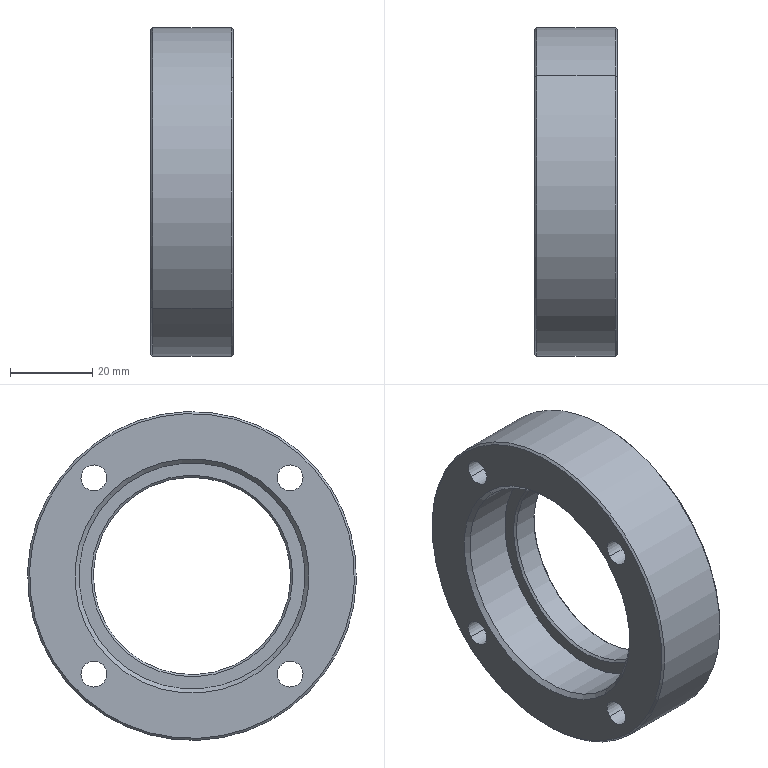Component | SolidWorks | LowerSideBeltXG-XG1-1_GB6006BearingHousingXG-XG1-1 | 1 solid | 39 faces | box 20 x 80 x 80 mm | volume 52764 mm3 | cylinder 22 | cone 10 | plane 7 | commonest cylinder face diameters 11 x8 6.3 x8 80 x2 55 x2 48 x2
STEP:
#1=COLOUR_RGB('',0.7922,0.8196,0.9333);
#2=FILL_AREA_STYLE_COLOUR('',#1);
#3=FILL_AREA_STYLE('',(#2));
#4=SURFACE_STYLE_FILL_AREA(#3);
#5=SURFACE_SIDE_STYLE('',(#4));
#6=SURFACE_STYLE_USAGE(.BOTH.,#5);
#7=PRESENTATION_STYLE_ASSIGNMENT((#6));
#8=CARTESIAN_POINT('',(-12.41,25.372,5.254));
#9=VERTEX_POINT('',#8);
#10=CARTESIAN_POINT('',(-12.41,23.841,3.723));
#11=VERTEX_POINT('',#10);
#12=CARTESIAN_POINT('',(-12.41,24.606,4.488));
#13=DIRECTION('',(-1.,-0.,-0.));
#14=DIRECTION('',(0.,-0.7071,-0.7071));
#15=AXIS2_PLACEMENT_3D('',#12,#13,#14);
#16=CIRCLE('',#15,1.083);
#17=EDGE_CURVE('',#9,#11,#16,.T.);
#18=ORIENTED_EDGE('',*,*,#17,.F.);
#19=CARTESIAN_POINT('',(-12.45,25.4,5.282));
#20=VERTEX_POINT('',#19);
#21=CARTESIAN_POINT('',(-12.45,25.4,5.282));
#22=DIRECTION('',(-0.7071,0.5,0.5));
#23=VECTOR('',#22,39.37);
#24=LINE('',#21,#23);
#25=EDGE_CURVE('',#9,#20,#24,.T.);
#26=ORIENTED_EDGE('',*,*,#25,.T.);
#27=CARTESIAN_POINT('',(-12.45,23.813,3.695));
#28=VERTEX_POINT('',#27);
#29=CARTESIAN_POINT('',(-12.45,24.606,4.488));
#30=DIRECTION('',(1.,0.,0.));
#31=DIRECTION('',(0.,-0.7071,-0.7071));
#32=AXIS2_PLACEMENT_3D('',#29,#30,#31);
#33=CIRCLE('',#32,1.122);
#34=EDGE_CURVE('',#28,#20,#33,.T.);
#35=ORIENTED_EDGE('',*,*,#34,.F.);
#36=CARTESIAN_POINT('',(-12.45,23.813,3.695));
#37=DIRECTION('',(-0.7071,-0.5,-0.5));
#38=VECTOR('',#37,39.37);
#39=LINE('',#36,#38);
#40=EDGE_CURVE('',#11,#28,#39,.T.);
#41=ORIENTED_EDGE('',*,*,#40,.F.);
#42=EDGE_LOOP('',(#18,#26,#35,#41));
#43=FACE_OUTER_BOUND('',#42,.T.);
#44=CARTESIAN_POINT('',(-12.45,24.606,4.488));
#45=DIRECTION('',(-1.,-0.,-0.));
#46=DIRECTION('',(0.,-0.7071,-0.7071));
#47=AXIS2_PLACEMENT_3D('',#44,#45,#46);
#48=CONICAL_SURFACE('',#47,1.122,0.7854);
#49=ADVANCED_FACE('',(#43),#48,.F.);
#50=CARTESIAN_POINT('',(-11.918,25.274,5.156));
#51=VERTEX_POINT('',#50);
#52=CARTESIAN_POINT('',(-11.918,23.938,3.82));
#53=VERTEX_POINT('',#52);
#54=CARTESIAN_POINT('',(-11.918,24.606,4.488));
#55=DIRECTION('',(-1.,-0.,-0.));
#56=DIRECTION('',(0.,-0.7071,-0.7071));
#57=AXIS2_PLACEMENT_3D('',#54,#55,#56);
#58=CIRCLE('',#57,0.9449);
#59=EDGE_CURVE('',#51,#53,#58,.T.);
#60=ORIENTED_EDGE('',*,*,#59,.F.);
#61=CARTESIAN_POINT('',(-11.938,25.288,5.17));
#62=VERTEX_POINT('',#61);
#63=CARTESIAN_POINT('',(-11.938,25.288,5.17));
#64=DIRECTION('',(-0.7071,0.5,0.5));
#65=VECTOR('',#64,39.37);
#66=LINE('',#63,#65);
#67=EDGE_CURVE('',#51,#62,#66,.T.);
#68=ORIENTED_EDGE('',*,*,#67,.T.);
#69=CARTESIAN_POINT('',(-11.938,23.924,3.806));
#70=VERTEX_POINT('',#69);
#71=CARTESIAN_POINT('',(-11.938,24.606,4.488));
#72=DIRECTION('',(1.,0.,0.));
#73=DIRECTION('',(0.,-0.7071,-0.7071));
#74=AXIS2_PLACEMENT_3D('',#71,#72,#73);
#75=CIRCLE('',#74,0.9646);
#76=EDGE_CURVE('',#70,#62,#75,.T.);
#77=ORIENTED_EDGE('',*,*,#76,.F.);
#78=CARTESIAN_POINT('',(-11.938,23.924,3.806));
#79=DIRECTION('',(-0.7071,-0.5,-0.5));
#80=VECTOR('',#79,39.37);
#81=LINE('',#78,#80);
#82=EDGE_CURVE('',#53,#70,#81,.T.);
#83=ORIENTED_EDGE('',*,*,#82,.F.);
#84=EDGE_LOOP('',(#60,#68,#77,#83));
#85=FACE_OUTER_BOUND('',#84,.T.);
#86=CARTESIAN_POINT('',(-11.938,24.606,4.488));
#87=DIRECTION('',(-1.,-0.,-0.));
#88=DIRECTION('',(0.,-0.7071,-0.7071));
#89=AXIS2_PLACEMENT_3D('',#86,#87,#88);
#90=CONICAL_SURFACE('',#89,0.9646,0.7854);
#91=ADVANCED_FACE('',(#85),#90,.F.);
#92=CARTESIAN_POINT('',(-11.682,23.938,3.82));
#93=VERTEX_POINT('',#92);
#94=CARTESIAN_POINT('',(-11.682,25.274,5.156));
#95=VERTEX_POINT('',#94);
#96=CARTESIAN_POINT('',(-11.682,24.606,4.488));
#97=DIRECTION('',(1.,0.,0.));
#98=DIRECTION('',(-0.,0.7071,0.7071));
#99=AXIS2_PLACEMENT_3D('',#96,#97,#98);
#100=CIRCLE('',#99,0.9449);
#101=EDGE_CURVE('',#93,#95,#100,.T.);
#102=ORIENTED_EDGE('',*,*,#101,.F.);
#103=CARTESIAN_POINT('',(-11.662,23.924,3.806));
#104=VERTEX_POINT('',#103);
#105=CARTESIAN_POINT('',(-11.682,23.938,3.82));
#106=DIRECTION('',(0.7071,-0.5,-0.5));
#107=VECTOR('',#106,39.37);
#108=LINE('',#105,#107);
#109=EDGE_CURVE('',#93,#104,#108,.T.);
#110=ORIENTED_EDGE('',*,*,#109,.T.);
#111=CARTESIAN_POINT('',(-11.662,25.288,5.17));
#112=VERTEX_POINT('',#111);
#113=CARTESIAN_POINT('',(-11.662,24.606,4.488));
#114=DIRECTION('',(-1.,-0.,-0.));
#115=DIRECTION('',(-0.,0.7071,0.7071));
#116=AXIS2_PLACEMENT_3D('',#113,#114,#115);
#117=CIRCLE('',#116,0.9646);
#118=EDGE_CURVE('',#112,#104,#117,.T.);
#119=ORIENTED_EDGE('',*,*,#118,.F.);
#120=CARTESIAN_POINT('',(-11.682,25.274,5.156));
#121=DIRECTION('',(0.7071,0.5,0.5));
#122=VECTOR('',#121,39.37);
#123=LINE('',#120,#122);
#124=EDGE_CURVE('',#95,#112,#123,.T.);
#125=ORIENTED_EDGE('',*,*,#124,.F.);
#126=EDGE_LOOP('',(#102,#110,#119,#125));
#127=FACE_OUTER_BOUND('',#126,.T.);
#128=CARTESIAN_POINT('',(-11.682,24.606,4.488));
#129=DIRECTION('',(1.,0.,0.));
#130=DIRECTION('',(-0.,0.7071,0.7071));
#131=AXIS2_PLACEMENT_3D('',#128,#129,#130);
#132=CONICAL_SURFACE('',#131,0.9449,0.7854);
#133=ADVANCED_FACE('',(#127),#132,.F.);
#134=CARTESIAN_POINT('',(-11.662,25.706,5.588));
#135=VERTEX_POINT('',#134);
#136=CARTESIAN_POINT('',(-11.662,23.507,3.389));
#137=VERTEX_POINT('',#136);
#138=CARTESIAN_POINT('',(-11.662,24.606,4.488));
#139=DIRECTION('',(1.,0.,0.));
#140=DIRECTION('',(-0.,0.7071,0.7071));
#141=AXIS2_PLACEMENT_3D('',#138,#139,#140);
#142=CIRCLE('',#141,1.555);
#143=EDGE_CURVE('',#135,#137,#142,.T.);
#144=ORIENTED_EDGE('',*,*,#143,.F.);
#145=CARTESIAN_POINT('',(-11.682,25.72,5.602));
#146=VERTEX_POINT('',#145);
#147=CARTESIAN_POINT('',(-11.662,25.706,5.588));
#148=DIRECTION('',(-0.7071,0.5,0.5));
#149=VECTOR('',#148,39.37);
#150=LINE('',#147,#149);
#151=EDGE_CURVE('',#135,#146,#150,.T.);
#152=ORIENTED_EDGE('',*,*,#151,.T.);
#153=CARTESIAN_POINT('',(-11.682,23.493,3.375));
#154=VERTEX_POINT('',#153);
#155=CARTESIAN_POINT('',(-11.682,24.606,4.488));
#156=DIRECTION('',(-1.,-0.,-0.));
#157=DIRECTION('',(-0.,0.7071,0.7071));
#158=AXIS2_PLACEMENT_3D('',#155,#156,#157);
#159=CIRCLE('',#158,1.575);
#160=EDGE_CURVE('',#154,#146,#159,.T.);
#161=ORIENTED_EDGE('',*,*,#160,.F.);
#162=CARTESIAN_POINT('',(-11.662,23.507,3.389));
#163=DIRECTION('',(-0.7071,-0.5,-0.5));
#164=VECTOR('',#163,39.37);
#165=LINE('',#162,#164);
#166=EDGE_CURVE('',#137,#154,#165,.T.);
#167=ORIENTED_EDGE('',*,*,#166,.F.);
#168=EDGE_LOOP('',(#144,#152,#161,#167));
#169=FACE_OUTER_BOUND('',#168,.T.);
#170=CARTESIAN_POINT('',(-11.662,24.606,4.488));
#171=DIRECTION('',(-1.,-0.,-0.));
#172=DIRECTION('',(0.,-0.7071,-0.7071));
#173=AXIS2_PLACEMENT_3D('',#170,#171,#172);
#174=CONICAL_SURFACE('',#173,1.555,0.7854);
#175=ADVANCED_FACE('',(#169),#174,.T.);
#176=CARTESIAN_POINT('',(-12.45,23.507,3.389));
#177=VERTEX_POINT('',#176);
#178=CARTESIAN_POINT('',(-12.45,25.706,5.588));
#179=VERTEX_POINT('',#178);
#180=CARTESIAN_POINT('',(-12.45,24.606,4.488));
#181=DIRECTION('',(-1.,-0.,-0.));
#182=DIRECTION('',(0.,-0.7071,-0.7071));
#183=AXIS2_PLACEMENT_3D('',#180,#181,#182);
#184=CIRCLE('',#183,1.555);
#185=EDGE_CURVE('',#177,#179,#184,.T.);
#186=ORIENTED_EDGE('',*,*,#185,.F.);
#187=CARTESIAN_POINT('',(-12.43,23.493,3.375));
#188=VERTEX_POINT('',#187);
#189=CARTESIAN_POINT('',(-12.43,23.493,3.375));
#190=DIRECTION('',(0.7071,-0.5,-0.5));
#191=VECTOR('',#190,39.37);
#192=LINE('',#189,#191);
#193=EDGE_CURVE('',#177,#188,#192,.T.);
#194=ORIENTED_EDGE('',*,*,#193,.T.);
#195=CARTESIAN_POINT('',(-12.43,25.72,5.602));
#196=VERTEX_POINT('',#195);
#197=CARTESIAN_POINT('',(-12.43,24.606,4.488));
#198=DIRECTION('',(1.,0.,0.));
#199=DIRECTION('',(0.,-0.7071,-0.7071));
#200=AXIS2_PLACEMENT_3D('',#197,#198,#199);
#201=CIRCLE('',#200,1.575);
#202=EDGE_CURVE('',#196,#188,#201,.T.);
#203=ORIENTED_EDGE('',*,*,#202,.F.);
#204=CARTESIAN_POINT('',(-12.43,25.72,5.602));
#205=DIRECTION('',(0.7071,0.5,0.5));
#206=VECTOR('',#205,39.37);
#207=LINE('',#204,#206);
#208=EDGE_CURVE('',#179,#196,#207,.T.);
#209=ORIENTED_EDGE('',*,*,#208,.F.);
#210=EDGE_LOOP('',(#186,#194,#203,#209));
#211=FACE_OUTER_BOUND('',#210,.T.);
#212=CARTESIAN_POINT('',(-12.43,24.606,4.488));
#213=DIRECTION('',(1.,0.,0.));
#214=DIRECTION('',(-0.,0.7071,0.7071));
#215=AXIS2_PLACEMENT_3D('',#212,#213,#214);
#216=CONICAL_SURFACE('',#215,1.575,0.7854);
#217=ADVANCED_FACE('',(#211),#216,.T.);
#218=CARTESIAN_POINT('',(-11.898,25.393,3.702));
#219=VERTEX_POINT('',#218);
#220=CARTESIAN_POINT('',(-11.898,25.699,3.396));
#221=VERTEX_POINT('',#220);
#222=CARTESIAN_POINT('',(-11.898,25.546,3.549));
#223=DIRECTION('',(1.,0.,-0.));
#224=DIRECTION('',(0.,0.7071,-0.7071));
#225=AXIS2_PLACEMENT_3D('',#222,#223,#224);
#226=CIRCLE('',#225,0.2165);
#227=EDGE_CURVE('',#219,#221,#226,.T.);
#228=ORIENTED_EDGE('',*,*,#227,.F.);
#229=CARTESIAN_POINT('',(-11.662,25.393,3.702));
#230=VERTEX_POINT('',#229);
#231=CARTESIAN_POINT('',(-11.662,25.393,3.702));
#232=DIRECTION('',(1.,0.,-0.));
#233=VECTOR('',#232,39.37);
#234=LINE('',#231,#233);
#235=EDGE_CURVE('',#219,#230,#234,.T.);
#236=ORIENTED_EDGE('',*,*,#235,.T.);
#237=CARTESIAN_POINT('',(-11.662,25.699,3.396));
#238=VERTEX_POINT('',#237);
#239=CARTESIAN_POINT('',(-11.662,25.546,3.549));
#240=DIRECTION('',(1.,0.,-0.));
#241=DIRECTION('',(0.,0.7071,-0.7071));
#242=AXIS2_PLACEMENT_3D('',#239,#240,#241);
#243=CIRCLE('',#242,0.2165);
#244=EDGE_CURVE('',#230,#238,#243,.T.);
#245=ORIENTED_EDGE('',*,*,#244,.T.);
#246=CARTESIAN_POINT('',(-11.662,25.699,3.396));
#247=DIRECTION('',(1.,0.,-0.));
#248=VECTOR('',#247,39.37);
#249=LINE('',#246,#248);
#250=EDGE_CURVE('',#221,#238,#249,.T.);
#251=ORIENTED_EDGE('',*,*,#250,.F.);
#252=EDGE_LOOP('',(#228,#236,#245,#251));
#253=FACE_OUTER_BOUND('',#252,.T.);
#254=CARTESIAN_POINT('',(-11.662,25.546,3.549));
#255=DIRECTION('',(1.,0.,-0.));
#256=DIRECTION('',(0.,0.7071,-0.7071));
#257=AXIS2_PLACEMENT_3D('',#254,#255,#256);
#258=CYLINDRICAL_SURFACE('',#257,0.2165);
#259=ADVANCED_FACE('',(#253),#258,.F.);
#260=CARTESIAN_POINT('',(-12.45,25.458,3.636));
#261=VERTEX_POINT('',#260);
#262=CARTESIAN_POINT('',(-12.45,25.634,3.461));
#263=VERTEX_POINT('',#262);
#264=CARTESIAN_POINT('',(-12.45,25.546,3.549));
#265=DIRECTION('',(1.,0.,-0.));
#266=DIRECTION('',(0.,0.7071,-0.7071));
#267=AXIS2_PLACEMENT_3D('',#264,#265,#266);
#268=CIRCLE('',#267,0.124);
#269=EDGE_CURVE('',#261,#263,#268,.T.);
#270=ORIENTED_EDGE('',*,*,#269,.F.);
#271=CARTESIAN_POINT('',(-11.898,25.458,3.636));
#272=VERTEX_POINT('',#271);
#273=CARTESIAN_POINT('',(-11.662,25.458,3.636));
#274=DIRECTION('',(1.,0.,-0.));
#275=VECTOR('',#274,39.37);
#276=LINE('',#273,#275);
#277=EDGE_CURVE('',#261,#272,#276,.T.);
#278=ORIENTED_EDGE('',*,*,#277,.T.);
#279=CARTESIAN_POINT('',(-11.898,25.634,3.461));
#280=VERTEX_POINT('',#279);
#281=CARTESIAN_POINT('',(-11.898,25.546,3.549));
#282=DIRECTION('',(1.,0.,-0.));
#283=DIRECTION('',(0.,0.7071,-0.7071));
#284=AXIS2_PLACEMENT_3D('',#281,#282,#283);
#285=CIRCLE('',#284,0.124);
#286=EDGE_CURVE('',#272,#280,#285,.T.);
#287=ORIENTED_EDGE('',*,*,#286,.T.);
#288=CARTESIAN_POINT('',(-11.662,25.634,3.461));
#289=DIRECTION('',(1.,0.,-0.));
#290=VECTOR('',#289,39.37);
#291=LINE('',#288,#290);
#292=EDGE_CURVE('',#263,#280,#291,.T.);
#293=ORIENTED_EDGE('',*,*,#292,.F.);
#294=EDGE_LOOP('',(#270,#278,#287,#293));
#295=FACE_OUTER_BOUND('',#294,.T.);
#296=CARTESIAN_POINT('',(-11.662,25.546,3.549));
#297=DIRECTION('',(1.,0.,-0.));
#298=DIRECTION('',(0.,0.7071,-0.7071));
#299=AXIS2_PLACEMENT_3D('',#296,#297,#298);
#300=CYLINDRICAL_SURFACE('',#299,0.124);
#301=ADVANCED_FACE('',(#295),#300,.F.);
#302=CARTESIAN_POINT('',(-11.898,25.393,5.581));
#303=VERTEX_POINT('',#302);
#304=CARTESIAN_POINT('',(-11.898,25.699,5.275));
#305=VERTEX_POINT('',#304);
#306=CARTESIAN_POINT('',(-11.898,25.546,5.428));
#307=DIRECTION('',(1.,0.,-0.));
#308=DIRECTION('',(0.,0.7071,-0.7071));
#309=AXIS2_PLACEMENT_3D('',#306,#307,#308);
#310=CIRCLE('',#309,0.2165);
#311=EDGE_CURVE('',#303,#305,#310,.T.);
#312=ORIENTED_EDGE('',*,*,#311,.F.);
#313=CARTESIAN_POINT('',(-11.662,25.393,5.581));
#314=VERTEX_POINT('',#313);
#315=CARTESIAN_POINT('',(-11.662,25.393,5.581));
#316=DIRECTION('',(1.,0.,-0.));
#317=VECTOR('',#316,39.37);
#318=LINE('',#315,#317);
#319=EDGE_CURVE('',#303,#314,#318,.T.);
#320=ORIENTED_EDGE('',*,*,#319,.T.);
#321=CARTESIAN_POINT('',(-11.662,25.699,5.275));
#322=VERTEX_POINT('',#321);
#323=CARTESIAN_POINT('',(-11.662,25.546,5.428));
#324=DIRECTION('',(1.,0.,-0.));
#325=DIRECTION('',(0.,0.7071,-0.7071));
#326=AXIS2_PLACEMENT_3D('',#323,#324,#325);
#327=CIRCLE('',#326,0.2165);
#328=EDGE_CURVE('',#314,#322,#327,.T.);
#329=ORIENTED_EDGE('',*,*,#328,.T.);
#330=CARTESIAN_POINT('',(-11.662,25.699,5.275));
#331=DIRECTION('',(1.,0.,-0.));
#332=VECTOR('',#331,39.37);
#333=LINE('',#330,#332);
#334=EDGE_CURVE('',#305,#322,#333,.T.);
#335=ORIENTED_EDGE('',*,*,#334,.F.);
#336=EDGE_LOOP('',(#312,#320,#329,#335));
#337=FACE_OUTER_BOUND('',#336,.T.);
#338=CARTESIAN_POINT('',(-11.662,25.546,5.428));
#339=DIRECTION('',(1.,0.,-0.));
#340=DIRECTION('',(0.,0.7071,-0.7071));
#341=AXIS2_PLACEMENT_3D('',#338,#339,#340);
#342=CYLINDRICAL_SURFACE('',#341,0.2165);
#343=ADVANCED_FACE('',(#337),#342,.F.);
#344=CARTESIAN_POINT('',(-12.45,25.458,5.515));
#345=VERTEX_POINT('',#344);
#346=CARTESIAN_POINT('',(-12.45,25.634,5.34));
#347=VERTEX_POINT('',#346);
#348=CARTESIAN_POINT('',(-12.45,25.546,5.428));
#349=DIRECTION('',(1.,0.,-0.));
#350=DIRECTION('',(0.,0.7071,-0.7071));
#351=AXIS2_PLACEMENT_3D('',#348,#349,#350);
#352=CIRCLE('',#351,0.124);
#353=EDGE_CURVE('',#345,#347,#352,.T.);
#354=ORIENTED_EDGE('',*,*,#353,.F.);
#355=CARTESIAN_POINT('',(-11.898,25.458,5.515));
#356=VERTEX_POINT('',#355);
#357=CARTESIAN_POINT('',(-11.662,25.458,5.515));
#358=DIRECTION('',(1.,0.,-0.));
#359=VECTOR('',#358,39.37);
#360=LINE('',#357,#359);
#361=EDGE_CURVE('',#345,#356,#360,.T.);
#362=ORIENTED_EDGE('',*,*,#361,.T.);
#363=CARTESIAN_POINT('',(-11.898,25.634,5.34));
#364=VERTEX_POINT('',#363);
#365=CARTESIAN_POINT('',(-11.898,25.546,5.428));
#366=DIRECTION('',(1.,0.,-0.));
#367=DIRECTION('',(0.,0.7071,-0.7071));
#368=AXIS2_PLACEMENT_3D('',#365,#366,#367);
#369=CIRCLE('',#368,0.124);
#370=EDGE_CURVE('',#356,#364,#369,.T.);
#371=ORIENTED_EDGE('',*,*,#370,.T.);
#372=CARTESIAN_POINT('',(-11.662,25.634,5.34));
#373=DIRECTION('',(1.,0.,-0.));
#374=VECTOR('',#373,39.37);
#375=LINE('',#372,#374);
#376=EDGE_CURVE('',#347,#364,#375,.T.);
#377=ORIENTED_EDGE('',*,*,#376,.F.);
#378=EDGE_LOOP('',(#354,#362,#371,#377));
#379=FACE_OUTER_BOUND('',#378,.T.);
#380=CARTESIAN_POINT('',(-11.662,25.546,5.428));
#381=DIRECTION('',(1.,0.,-0.));
#382=DIRECTION('',(0.,0.7071,-0.7071));
#383=AXIS2_PLACEMENT_3D('',#380,#381,#382);
#384=CYLINDRICAL_SURFACE('',#383,0.124);
#385=ADVANCED_FACE('',(#379),#384,.F.);
#386=CARTESIAN_POINT('',(-11.898,23.514,3.702));
#387=VERTEX_POINT('',#386);
#388=CARTESIAN_POINT('',(-11.898,23.82,3.396));
#389=VERTEX_POINT('',#388);
#390=CARTESIAN_POINT('',(-11.898,23.667,3.549));
#391=DIRECTION('',(1.,0.,-0.));
#392=DIRECTION('',(0.,0.7071,-0.7071));
#393=AXIS2_PLACEMENT_3D('',#390,#391,#392);
#394=CIRCLE('',#393,0.2165);
#395=EDGE_CURVE('',#387,#389,#394,.T.);
#396=ORIENTED_EDGE('',*,*,#395,.F.);
#397=CARTESIAN_POINT('',(-11.662,23.514,3.702));
#398=VERTEX_POINT('',#397);
#399=CARTESIAN_POINT('',(-11.662,23.514,3.702));
#400=DIRECTION('',(1.,0.,-0.));
#401=VECTOR('',#400,39.37);
#402=LINE('',#399,#401);
#403=EDGE_CURVE('',#387,#398,#402,.T.);
#404=ORIENTED_EDGE('',*,*,#403,.T.);
#405=CARTESIAN_POINT('',(-11.662,23.82,3.396));
#406=VERTEX_POINT('',#405);
#407=CARTESIAN_POINT('',(-11.662,23.667,3.549));
#408=DIRECTION('',(1.,0.,-0.));
#409=DIRECTION('',(0.,0.7071,-0.7071));
#410=AXIS2_PLACEMENT_3D('',#407,#408,#409);
#411=CIRCLE('',#410,0.2165);
#412=EDGE_CURVE('',#398,#406,#411,.T.);
#413=ORIENTED_EDGE('',*,*,#412,.T.);
#414=CARTESIAN_POINT('',(-11.662,23.82,3.396));
#415=DIRECTION('',(1.,0.,-0.));
#416=VECTOR('',#415,39.37);
#417=LINE('',#414,#416);
#418=EDGE_CURVE('',#389,#406,#417,.T.);
#419=ORIENTED_EDGE('',*,*,#418,.F.);
#420=EDGE_LOOP('',(#396,#404,#413,#419));
#421=FACE_OUTER_BOUND('',#420,.T.);
#422=CARTESIAN_POINT('',(-11.662,23.667,3.549));
#423=DIRECTION('',(1.,0.,-0.));
#424=DIRECTION('',(0.,0.7071,-0.7071));
#425=AXIS2_PLACEMENT_3D('',#422,#423,#424);
#426=CYLINDRICAL_SURFACE('',#425,0.2165);
#427=ADVANCED_FACE('',(#421),#426,.F.);
#428=CARTESIAN_POINT('',(-12.45,23.579,3.636));
#429=VERTEX_POINT('',#428);
#430=CARTESIAN_POINT('',(-12.45,23.754,3.461));
#431=VERTEX_POINT('',#430);
#432=CARTESIAN_POINT('',(-12.45,23.667,3.549));
#433=DIRECTION('',(1.,0.,-0.));
#434=DIRECTION('',(0.,0.7071,-0.7071));
#435=AXIS2_PLACEMENT_3D('',#432,#433,#434);
#436=CIRCLE('',#435,0.124);
#437=EDGE_CURVE('',#429,#431,#436,.T.);
#438=ORIENTED_EDGE('',*,*,#437,.F.);
#439=CARTESIAN_POINT('',(-11.898,23.579,3.636));
#440=VERTEX_POINT('',#439);
#441=CARTESIAN_POINT('',(-11.662,23.579,3.636));
#442=DIRECTION('',(1.,0.,-0.));
#443=VECTOR('',#442,39.37);
#444=LINE('',#441,#443);
#445=EDGE_CURVE('',#429,#440,#444,.T.);
#446=ORIENTED_EDGE('',*,*,#445,.T.);
#447=CARTESIAN_POINT('',(-11.898,23.754,3.461));
#448=VERTEX_POINT('',#447);
#449=CARTESIAN_POINT('',(-11.898,23.667,3.549));
#450=DIRECTION('',(1.,0.,-0.));
#451=DIRECTION('',(0.,0.7071,-0.7071));
#452=AXIS2_PLACEMENT_3D('',#449,#450,#451);
#453=CIRCLE('',#452,0.124);
#454=EDGE_CURVE('',#440,#448,#453,.T.);
#455=ORIENTED_EDGE('',*,*,#454,.T.);
#456=CARTESIAN_POINT('',(-11.662,23.754,3.461));
#457=DIRECTION('',(1.,0.,-0.));
#458=VECTOR('',#457,39.37);
#459=LINE('',#456,#458);
#460=EDGE_CURVE('',#431,#448,#459,.T.);
#461=ORIENTED_EDGE('',*,*,#460,.F.);
#462=EDGE_LOOP('',(#438,#446,#455,#461));
#463=FACE_OUTER_BOUND('',#462,.T.);
#464=CARTESIAN_POINT('',(-11.662,23.667,3.549));
#465=DIRECTION('',(1.,0.,-0.));
#466=DIRECTION('',(0.,0.7071,-0.7071));
#467=AXIS2_PLACEMENT_3D('',#464,#465,#466);
#468=CYLINDRICAL_SURFACE('',#467,0.124);
#469=ADVANCED_FACE('',(#463),#468,.F.);
#470=CARTESIAN_POINT('',(-11.898,23.514,5.581));
#471=VERTEX_POINT('',#470);
#472=CARTESIAN_POINT('',(-11.898,23.82,5.275));
#473=VERTEX_POINT('',#472);
#474=CARTESIAN_POINT('',(-11.898,23.667,5.428));
#475=DIRECTION('',(1.,0.,-0.));
#476=DIRECTION('',(0.,0.7071,-0.7071));
#477=AXIS2_PLACEMENT_3D('',#474,#475,#476);
#478=CIRCLE('',#477,0.2165);
#479=EDGE_CURVE('',#471,#473,#478,.T.);
#480=ORIENTED_EDGE('',*,*,#479,.F.);
#481=CARTESIAN_POINT('',(-11.662,23.514,5.581));
#482=VERTEX_POINT('',#481);
#483=CARTESIAN_POINT('',(-11.662,23.514,5.581));
#484=DIRECTION('',(1.,0.,-0.));
#485=VECTOR('',#484,39.37);
#486=LINE('',#483,#485);
#487=EDGE_CURVE('',#471,#482,#486,.T.);
#488=ORIENTED_EDGE('',*,*,#487,.T.);
#489=CARTESIAN_POINT('',(-11.662,23.82,5.275));
#490=VERTEX_POINT('',#489);
#491=CARTESIAN_POINT('',(-11.662,23.667,5.428));
#492=DIRECTION('',(1.,0.,-0.));
#493=DIRECTION('',(0.,0.7071,-0.7071));
#494=AXIS2_PLACEMENT_3D('',#491,#492,#493);
#495=CIRCLE('',#494,0.2165);
#496=EDGE_CURVE('',#482,#490,#495,.T.);
#497=ORIENTED_EDGE('',*,*,#496,.T.);
#498=CARTESIAN_POINT('',(-11.662,23.82,5.275));
#499=DIRECTION('',(1.,0.,-0.));
#500=VECTOR('',#499,39.37);
#501=LINE('',#498,#500);
#502=EDGE_CURVE('',#473,#490,#501,.T.);
#503=ORIENTED_EDGE('',*,*,#502,.F.);
#504=EDGE_LOOP('',(#480,#488,#497,#503));
#505=FACE_OUTER_BOUND('',#504,.T.);
#506=CARTESIAN_POINT('',(-11.662,23.667,5.428));
#507=DIRECTION('',(1.,0.,-0.));
#508=DIRECTION('',(0.,0.7071,-0.7071));
#509=AXIS2_PLACEMENT_3D('',#506,#507,#508);
#510=CYLINDRICAL_SURFACE('',#509,0.2165);
#511=ADVANCED_FACE('',(#505),#510,.F.);
#512=CARTESIAN_POINT('',(-12.45,23.579,5.515));
#513=VERTEX_POINT('',#512);
#514=CARTESIAN_POINT('',(-12.45,23.754,5.34));
#515=VERTEX_POINT('',#514);
#516=CARTESIAN_POINT('',(-12.45,23.667,5.428));
#517=DIRECTION('',(1.,0.,-0.));
#518=DIRECTION('',(0.,0.7071,-0.7071));
#519=AXIS2_PLACEMENT_3D('',#516,#517,#518);
#520=CIRCLE('',#519,0.124);
#521=EDGE_CURVE('',#513,#515,#520,.T.);
#522=ORIENTED_EDGE('',*,*,#521,.F.);
#523=CARTESIAN_POINT('',(-11.898,23.579,5.515));
#524=VERTEX_POINT('',#523);
#525=CARTESIAN_POINT('',(-11.662,23.579,5.515));
#526=DIRECTION('',(1.,0.,-0.));
#527=VECTOR('',#526,39.37);
#528=LINE('',#525,#527);
#529=EDGE_CURVE('',#513,#524,#528,.T.);
#530=ORIENTED_EDGE('',*,*,#529,.T.);
#531=CARTESIAN_POINT('',(-11.898,23.754,5.34));
#532=VERTEX_POINT('',#531);
#533=CARTESIAN_POINT('',(-11.898,23.667,5.428));
#534=DIRECTION('',(1.,0.,-0.));
#535=DIRECTION('',(0.,0.7071,-0.7071));
#536=AXIS2_PLACEMENT_3D('',#533,#534,#535);
#537=CIRCLE('',#536,0.124);
#538=EDGE_CURVE('',#524,#532,#537,.T.);
#539=ORIENTED_EDGE('',*,*,#538,.T.);
#540=CARTESIAN_POINT('',(-11.662,23.754,5.34));
#541=DIRECTION('',(1.,0.,-0.));
#542=VECTOR('',#541,39.37);
#543=LINE('',#540,#542);
#544=EDGE_CURVE('',#515,#532,#543,.T.);
#545=ORIENTED_EDGE('',*,*,#544,.F.);
#546=EDGE_LOOP('',(#522,#530,#539,#545));
#547=FACE_OUTER_BOUND('',#546,.T.);
#548=CARTESIAN_POINT('',(-11.662,23.667,5.428));
#549=DIRECTION('',(1.,0.,-0.));
#550=DIRECTION('',(0.,0.7071,-0.7071));
#551=AXIS2_PLACEMENT_3D('',#548,#549,#550);
#552=CYLINDRICAL_SURFACE('',#551,0.124);
#553=ADVANCED_FACE('',(#547),#552,.F.);
#554=ORIENTED_EDGE('',*,*,#202,.T.);
#555=CARTESIAN_POINT('',(8.65,23.493,3.375));
#556=DIRECTION('',(1.,0.,0.));
#557=VECTOR('',#556,39.37);
#558=LINE('',#555,#557);
#559=EDGE_CURVE('',#188,#154,#558,.T.);
#560=ORIENTED_EDGE('',*,*,#559,.T.);
#561=ORIENTED_EDGE('',*,*,#160,.T.);
#562=CARTESIAN_POINT('',(8.65,25.72,5.602));
#563=DIRECTION('',(1.,0.,0.));
#564=VECTOR('',#563,39.37);
#565=LINE('',#562,#564);
#566=EDGE_CURVE('',#196,#146,#565,.T.);
#567=ORIENTED_EDGE('',*,*,#566,.F.);
#568=EDGE_LOOP('',(#554,#560,#561,#567));
#569=FACE_OUTER_BOUND('',#568,.T.);
#570=CARTESIAN_POINT('',(8.65,24.606,4.488));
#571=DIRECTION('',(1.,0.,0.));
#572=DIRECTION('',(-0.,0.7071,0.7071));
#573=AXIS2_PLACEMENT_3D('',#570,#571,#572);
#574=CYLINDRICAL_SURFACE('',#573,1.575);
#575=ADVANCED_FACE('',(#569),#574,.T.);
#576=ORIENTED_EDGE('',*,*,#17,.T.);
#577=CARTESIAN_POINT('',(-11.938,23.841,3.723));
#578=VERTEX_POINT('',#577);
#579=CARTESIAN_POINT('',(8.65,23.841,3.723));
#580=DIRECTION('',(1.,0.,0.));
#581=VECTOR('',#580,39.37);
#582=LINE('',#579,#581);
#583=EDGE_CURVE('',#11,#578,#582,.T.);
#584=ORIENTED_EDGE('',*,*,#583,.T.);
#585=CARTESIAN_POINT('',(-11.938,25.372,5.254));
#586=VERTEX_POINT('',#585);
#587=CARTESIAN_POINT('',(-11.938,24.606,4.488));
#588=DIRECTION('',(1.,0.,0.));
#589=DIRECTION('',(-0.,0.7071,0.7071));
#590=AXIS2_PLACEMENT_3D('',#587,#588,#589);
#591=CIRCLE('',#590,1.083);
#592=EDGE_CURVE('',#578,#586,#591,.T.);
#593=ORIENTED_EDGE('',*,*,#592,.T.);
#594=CARTESIAN_POINT('',(8.65,25.372,5.254));
#595=DIRECTION('',(1.,0.,0.));
#596=VECTOR('',#595,39.37);
#597=LINE('',#594,#596);
#598=EDGE_CURVE('',#9,#586,#597,.T.);
#599=ORIENTED_EDGE('',*,*,#598,.F.);
#600=EDGE_LOOP('',(#576,#584,#593,#599));
#601=FACE_OUTER_BOUND('',#600,.T.);
#602=CARTESIAN_POINT('',(8.65,24.606,4.488));
#603=DIRECTION('',(1.,0.,0.));
#604=DIRECTION('',(-0.,0.7071,0.7071));
#605=AXIS2_PLACEMENT_3D('',#602,#603,#604);
#606=CYLINDRICAL_SURFACE('',#605,1.083);
#607=ADVANCED_FACE('',(#601),#606,.F.);
#608=ORIENTED_EDGE('',*,*,#59,.T.);
#609=CARTESIAN_POINT('',(8.65,23.938,3.82));
#610=DIRECTION('',(1.,0.,0.));
#611=VECTOR('',#610,39.37);
#612=LINE('',#609,#611);
#613=EDGE_CURVE('',#53,#93,#612,.T.);
#614=ORIENTED_EDGE('',*,*,#613,.T.);
#615=ORIENTED_EDGE('',*,*,#101,.T.);
#616=CARTESIAN_POINT('',(8.65,25.274,5.156));
#617=DIRECTION('',(1.,0.,0.));
#618=VECTOR('',#617,39.37);
#619=LINE('',#616,#618);
#620=EDGE_CURVE('',#51,#95,#619,.T.);
#621=ORIENTED_EDGE('',*,*,#620,.F.);
#622=EDGE_LOOP('',(#608,#614,#615,#621));
#623=FACE_OUTER_BOUND('',#622,.T.);
#624=CARTESIAN_POINT('',(8.65,24.606,4.488));
#625=DIRECTION('',(1.,0.,0.));
#626=DIRECTION('',(-0.,0.7071,0.7071));
#627=AXIS2_PLACEMENT_3D('',#624,#625,#626);
#628=CYLINDRICAL_SURFACE('',#627,0.9449);
#629=ADVANCED_FACE('',(#623),#628,.F.);
#630=ORIENTED_EDGE('',*,*,#34,.T.);
#631=CARTESIAN_POINT('',(-12.45,24.606,4.488));
#632=DIRECTION('',(1.,0.,0.));
#633=DIRECTION('',(0.,-0.7071,-0.7071));
#634=AXIS2_PLACEMENT_3D('',#631,#632,#633);
#635=CIRCLE('',#634,1.122);
#636=EDGE_CURVE('',#20,#28,#635,.T.);
#637=ORIENTED_EDGE('',*,*,#636,.T.);
#638=EDGE_LOOP('',(#630,#637));
#639=FACE_BOUND('',#638,.T.);
#640=CARTESIAN_POINT('',(-12.45,24.606,4.488));
#641=DIRECTION('',(-1.,-0.,-0.));
#642=DIRECTION('',(0.,-0.7071,-0.7071));
#643=AXIS2_PLACEMENT_3D('',#640,#641,#642);
#644=CIRCLE('',#643,1.555);
#645=EDGE_CURVE('',#179,#177,#644,.T.);
#646=ORIENTED_EDGE('',*,*,#645,.T.);
#647=ORIENTED_EDGE('',*,*,#185,.T.);
#648=EDGE_LOOP('',(#646,#647));
#649=FACE_OUTER_BOUND('',#648,.T.);
#650=CARTESIAN_POINT('',(-12.45,23.667,5.428));
#651=DIRECTION('',(1.,0.,-0.));
#652=DIRECTION('',(0.,0.7071,-0.7071));
#653=AXIS2_PLACEMENT_3D('',#650,#651,#652);
#654=CIRCLE('',#653,0.124);
#655=EDGE_CURVE('',#515,#513,#654,.T.);
#656=ORIENTED_EDGE('',*,*,#655,.T.);
#657=ORIENTED_EDGE('',*,*,#521,.T.);
#658=EDGE_LOOP('',(#656,#657));
#659=FACE_BOUND('',#658,.T.);
#660=CARTESIAN_POINT('',(-12.45,23.667,3.549));
#661=DIRECTION('',(1.,0.,-0.));
#662=DIRECTION('',(0.,0.7071,-0.7071));
#663=AXIS2_PLACEMENT_3D('',#660,#661,#662);
#664=CIRCLE('',#663,0.124);
#665=EDGE_CURVE('',#431,#429,#664,.T.);
#666=ORIENTED_EDGE('',*,*,#665,.T.);
#667=ORIENTED_EDGE('',*,*,#437,.T.);
#668=EDGE_LOOP('',(#666,#667));
#669=FACE_BOUND('',#668,.T.);
#670=CARTESIAN_POINT('',(-12.45,25.546,5.428));
#671=DIRECTION('',(1.,0.,-0.));
#672=DIRECTION('',(0.,0.7071,-0.7071));
#673=AXIS2_PLACEMENT_3D('',#670,#671,#672);
#674=CIRCLE('',#673,0.124);
#675=EDGE_CURVE('',#347,#345,#674,.T.);
#676=ORIENTED_EDGE('',*,*,#675,.T.);
#677=ORIENTED_EDGE('',*,*,#353,.T.);
#678=EDGE_LOOP('',(#676,#677));
#679=FACE_BOUND('',#678,.T.);
#680=CARTESIAN_POINT('',(-12.45,25.546,3.549));
#681=DIRECTION('',(1.,0.,-0.));
#682=DIRECTION('',(0.,0.7071,-0.7071));
#683=AXIS2_PLACEMENT_3D('',#680,#681,#682);
#684=CIRCLE('',#683,0.124);
#685=EDGE_CURVE('',#263,#261,#684,.T.);
#686=ORIENTED_EDGE('',*,*,#685,.T.);
#687=ORIENTED_EDGE('',*,*,#269,.T.);
#688=EDGE_LOOP('',(#686,#687));
#689=FACE_BOUND('',#688,.T.);
#690=CARTESIAN_POINT('',(-12.45,25.372,5.254));
#691=DIRECTION('',(-1.,-0.,-0.));
#692=DIRECTION('',(0.,-0.7071,-0.7071));
#693=AXIS2_PLACEMENT_3D('',#690,#691,#692);
#694=PLANE('',#693);
#695=ADVANCED_FACE('',(#639,#649,#659,#669,#679,#689),#694,.T.);
#696=CARTESIAN_POINT('',(-11.662,24.606,4.488));
#697=DIRECTION('',(1.,0.,0.));
#698=DIRECTION('',(-0.,0.7071,0.7071));
#699=AXIS2_PLACEMENT_3D('',#696,#697,#698);
#700=CIRCLE('',#699,1.555);
#701=EDGE_CURVE('',#137,#135,#700,.T.);
#702=ORIENTED_EDGE('',*,*,#701,.T.);
#703=ORIENTED_EDGE('',*,*,#143,.T.);
#704=EDGE_LOOP('',(#702,#703));
#705=FACE_OUTER_BOUND('',#704,.T.);
#706=ORIENTED_EDGE('',*,*,#118,.T.);
#707=CARTESIAN_POINT('',(-11.662,24.606,4.488));
#708=DIRECTION('',(-1.,-0.,-0.));
#709=DIRECTION('',(-0.,0.7071,0.7071));
#710=AXIS2_PLACEMENT_3D('',#707,#708,#709);
#711=CIRCLE('',#710,0.9646);
#712=EDGE_CURVE('',#104,#112,#711,.T.);
#713=ORIENTED_EDGE('',*,*,#712,.T.);
#714=EDGE_LOOP('',(#706,#713));
#715=FACE_BOUND('',#714,.T.);
#716=CARTESIAN_POINT('',(-11.662,25.546,3.549));
#717=DIRECTION('',(1.,0.,-0.));
#718=DIRECTION('',(0.,0.7071,-0.7071));
#719=AXIS2_PLACEMENT_3D('',#716,#717,#718);
#720=CIRCLE('',#719,0.2165);
#721=EDGE_CURVE('',#238,#230,#720,.T.);
#722=ORIENTED_EDGE('',*,*,#721,.F.);
#723=ORIENTED_EDGE('',*,*,#244,.F.);
#724=EDGE_LOOP('',(#722,#723));
#725=FACE_BOUND('',#724,.T.);
#726=CARTESIAN_POINT('',(-11.662,25.546,5.428));
#727=DIRECTION('',(1.,0.,-0.));
#728=DIRECTION('',(0.,0.7071,-0.7071));
#729=AXIS2_PLACEMENT_3D('',#726,#727,#728);
#730=CIRCLE('',#729,0.2165);
#731=EDGE_CURVE('',#322,#314,#730,.T.);
#732=ORIENTED_EDGE('',*,*,#731,.F.);
#733=ORIENTED_EDGE('',*,*,#328,.F.);
#734=EDGE_LOOP('',(#732,#733));
#735=FACE_BOUND('',#734,.T.);
#736=CARTESIAN_POINT('',(-11.662,23.667,3.549));
#737=DIRECTION('',(1.,0.,-0.));
#738=DIRECTION('',(0.,0.7071,-0.7071));
#739=AXIS2_PLACEMENT_3D('',#736,#737,#738);
#740=CIRCLE('',#739,0.2165);
#741=EDGE_CURVE('',#406,#398,#740,.T.);
#742=ORIENTED_EDGE('',*,*,#741,.F.);
#743=ORIENTED_EDGE('',*,*,#412,.F.);
#744=EDGE_LOOP('',(#742,#743));
#745=FACE_BOUND('',#744,.T.);
#746=CARTESIAN_POINT('',(-11.662,23.667,5.428));
#747=DIRECTION('',(1.,0.,-0.));
#748=DIRECTION('',(0.,0.7071,-0.7071));
#749=AXIS2_PLACEMENT_3D('',#746,#747,#748);
#750=CIRCLE('',#749,0.2165);
#751=EDGE_CURVE('',#490,#482,#750,.T.);
#752=ORIENTED_EDGE('',*,*,#751,.F.);
#753=ORIENTED_EDGE('',*,*,#496,.F.);
#754=EDGE_LOOP('',(#752,#753));
#755=FACE_BOUND('',#754,.T.);
#756=CARTESIAN_POINT('',(-11.662,25.72,5.602));
#757=DIRECTION('',(1.,0.,0.));
#758=DIRECTION('',(-0.,0.7071,0.7071));
#759=AXIS2_PLACEMENT_3D('',#756,#757,#758);
#760=PLANE('',#759);
#761=ADVANCED_FACE('',(#705,#715,#725,#735,#745,#755),#760,.T.);
#762=ORIENTED_EDGE('',*,*,#613,.F.);
#763=CARTESIAN_POINT('',(-11.918,24.606,4.488));
#764=DIRECTION('',(-1.,-0.,-0.));
#765=DIRECTION('',(0.,-0.7071,-0.7071));
#766=AXIS2_PLACEMENT_3D('',#763,#764,#765);
#767=CIRCLE('',#766,0.9449);
#768=EDGE_CURVE('',#53,#51,#767,.T.);
#769=ORIENTED_EDGE('',*,*,#768,.T.);
#770=ORIENTED_EDGE('',*,*,#620,.T.);
#771=CARTESIAN_POINT('',(-11.682,24.606,4.488));
#772=DIRECTION('',(1.,0.,0.));
#773=DIRECTION('',(-0.,0.7071,0.7071));
#774=AXIS2_PLACEMENT_3D('',#771,#772,#773);
#775=CIRCLE('',#774,0.9449);
#776=EDGE_CURVE('',#95,#93,#775,.T.);
#777=ORIENTED_EDGE('',*,*,#776,.T.);
#778=EDGE_LOOP('',(#762,#769,#770,#777));
#779=FACE_OUTER_BOUND('',#778,.T.);
#780=CARTESIAN_POINT('',(8.65,24.606,4.488));
#781=DIRECTION('',(1.,0.,0.));
#782=DIRECTION('',(-0.,0.7071,0.7071));
#783=AXIS2_PLACEMENT_3D('',#780,#781,#782);
#784=CYLINDRICAL_SURFACE('',#783,0.9449);
#785=ADVANCED_FACE('',(#779),#784,.F.);
#786=ORIENTED_EDGE('',*,*,#76,.T.);
#787=CARTESIAN_POINT('',(-11.938,24.606,4.488));
#788=DIRECTION('',(1.,0.,0.));
#789=DIRECTION('',(0.,-0.7071,-0.7071));
#790=AXIS2_PLACEMENT_3D('',#787,#788,#789);
#791=CIRCLE('',#790,0.9646);
#792=EDGE_CURVE('',#62,#70,#791,.T.);
#793=ORIENTED_EDGE('',*,*,#792,.T.);
#794=EDGE_LOOP('',(#786,#793));
#795=FACE_BOUND('',#794,.T.);
#796=CARTESIAN_POINT('',(-11.938,24.606,4.488));
#797=DIRECTION('',(1.,0.,0.));
#798=DIRECTION('',(-0.,0.7071,0.7071));
#799=AXIS2_PLACEMENT_3D('',#796,#797,#798);
#800=CIRCLE('',#799,1.083);
#801=EDGE_CURVE('',#586,#578,#800,.T.);
#802=ORIENTED_EDGE('',*,*,#801,.F.);
#803=ORIENTED_EDGE('',*,*,#592,.F.);
#804=EDGE_LOOP('',(#802,#803));
#805=FACE_OUTER_BOUND('',#804,.T.);
#806=CARTESIAN_POINT('',(-11.938,25.274,5.156));
#807=DIRECTION('',(-1.,-0.,-0.));
#808=DIRECTION('',(0.,-0.7071,-0.7071));
#809=AXIS2_PLACEMENT_3D('',#806,#807,#808);
#810=PLANE('',#809);
#811=ADVANCED_FACE('',(#795,#805),#810,.T.);
#812=ORIENTED_EDGE('',*,*,#583,.F.);
#813=CARTESIAN_POINT('',(-12.41,24.606,4.488));
#814=DIRECTION('',(-1.,-0.,-0.));
#815=DIRECTION('',(0.,-0.7071,-0.7071));
#816=AXIS2_PLACEMENT_3D('',#813,#814,#815);
#817=CIRCLE('',#816,1.083);
#818=EDGE_CURVE('',#11,#9,#817,.T.);
#819=ORIENTED_EDGE('',*,*,#818,.T.);
#820=ORIENTED_EDGE('',*,*,#598,.T.);
#821=ORIENTED_EDGE('',*,*,#801,.T.);
#822=EDGE_LOOP('',(#812,#819,#820,#821));
#823=FACE_OUTER_BOUND('',#822,.T.);
#824=CARTESIAN_POINT('',(8.65,24.606,4.488));
#825=DIRECTION('',(1.,0.,0.));
#826=DIRECTION('',(-0.,0.7071,0.7071));
#827=AXIS2_PLACEMENT_3D('',#824,#825,#826);
#828=CYLINDRICAL_SURFACE('',#827,1.083);
#829=ADVANCED_FACE('',(#823),#828,.F.);
#830=ORIENTED_EDGE('',*,*,#559,.F.);
#831=CARTESIAN_POINT('',(-12.43,24.606,4.488));
#832=DIRECTION('',(1.,0.,0.));
#833=DIRECTION('',(0.,-0.7071,-0.7071));
#834=AXIS2_PLACEMENT_3D('',#831,#832,#833);
#835=CIRCLE('',#834,1.575);
#836=EDGE_CURVE('',#188,#196,#835,.T.);
#837=ORIENTED_EDGE('',*,*,#836,.T.);
#838=ORIENTED_EDGE('',*,*,#566,.T.);
#839=CARTESIAN_POINT('',(-11.682,24.606,4.488));
#840=DIRECTION('',(-1.,-0.,-0.));
#841=DIRECTION('',(-0.,0.7071,0.7071));
#842=AXIS2_PLACEMENT_3D('',#839,#840,#841);
#843=CIRCLE('',#842,1.575);
#844=EDGE_CURVE('',#146,#154,#843,.T.);
#845=ORIENTED_EDGE('',*,*,#844,.T.);
#846=EDGE_LOOP('',(#830,#837,#838,#845));
#847=FACE_OUTER_BOUND('',#846,.T.);
#848=CARTESIAN_POINT('',(8.65,24.606,4.488));
#849=DIRECTION('',(1.,0.,0.));
#850=DIRECTION('',(-0.,0.7071,0.7071));
#851=AXIS2_PLACEMENT_3D('',#848,#849,#850);
#852=CYLINDRICAL_SURFACE('',#851,1.575);
#853=ADVANCED_FACE('',(#847),#852,.T.);
#854=ORIENTED_EDGE('',*,*,#529,.F.);
#855=ORIENTED_EDGE('',*,*,#655,.F.);
#856=ORIENTED_EDGE('',*,*,#544,.T.);
#857=CARTESIAN_POINT('',(-11.898,23.667,5.428));
#858=DIRECTION('',(1.,0.,-0.));
#859=DIRECTION('',(0.,0.7071,-0.7071));
#860=AXIS2_PLACEMENT_3D('',#857,#858,#859);
#861=CIRCLE('',#860,0.124);
#862=EDGE_CURVE('',#532,#524,#861,.T.);
#863=ORIENTED_EDGE('',*,*,#862,.T.);
#864=EDGE_LOOP('',(#854,#855,#856,#863));
#865=FACE_OUTER_BOUND('',#864,.T.);
#866=CARTESIAN_POINT('',(-11.662,23.667,5.428));
#867=DIRECTION('',(1.,0.,-0.));
#868=DIRECTION('',(0.,0.7071,-0.7071));
#869=AXIS2_PLACEMENT_3D('',#866,#867,#868);
#870=CYLINDRICAL_SURFACE('',#869,0.124);
#871=ADVANCED_FACE('',(#865),#870,.F.);
#872=ORIENTED_EDGE('',*,*,#862,.F.);
#873=ORIENTED_EDGE('',*,*,#538,.F.);
#874=EDGE_LOOP('',(#872,#873));
#875=FACE_BOUND('',#874,.T.);
#876=CARTESIAN_POINT('',(-11.898,23.667,5.428));
#877=DIRECTION('',(1.,0.,-0.));
#878=DIRECTION('',(0.,0.7071,-0.7071));
#879=AXIS2_PLACEMENT_3D('',#876,#877,#878);
#880=CIRCLE('',#879,0.2165);
#881=EDGE_CURVE('',#473,#471,#880,.T.);
#882=ORIENTED_EDGE('',*,*,#881,.T.);
#883=ORIENTED_EDGE('',*,*,#479,.T.);
#884=EDGE_LOOP('',(#882,#883));
#885=FACE_OUTER_BOUND('',#884,.T.);
#886=CARTESIAN_POINT('',(-11.898,23.754,5.515));
#887=DIRECTION('',(-1.,-0.,-0.));
#888=DIRECTION('',(0.,-0.7071,0.7071));
#889=AXIS2_PLACEMENT_3D('',#886,#887,#888);
#890=PLANE('',#889);
#891=ADVANCED_FACE('',(#875,#885),#890,.F.);
#892=ORIENTED_EDGE('',*,*,#487,.F.);
#893=ORIENTED_EDGE('',*,*,#881,.F.);
#894=ORIENTED_EDGE('',*,*,#502,.T.);
#895=ORIENTED_EDGE('',*,*,#751,.T.);
#896=EDGE_LOOP('',(#892,#893,#894,#895));
#897=FACE_OUTER_BOUND('',#896,.T.);
#898=CARTESIAN_POINT('',(-11.662,23.667,5.428));
#899=DIRECTION('',(1.,0.,-0.));
#900=DIRECTION('',(0.,0.7071,-0.7071));
#901=AXIS2_PLACEMENT_3D('',#898,#899,#900);
#902=CYLINDRICAL_SURFACE('',#901,0.2165);
#903=ADVANCED_FACE('',(#897),#902,.F.);
#904=ORIENTED_EDGE('',*,*,#445,.F.);
#905=ORIENTED_EDGE('',*,*,#665,.F.);
#906=ORIENTED_EDGE('',*,*,#460,.T.);
#907=CARTESIAN_POINT('',(-11.898,23.667,3.549));
#908=DIRECTION('',(1.,0.,-0.));
#909=DIRECTION('',(0.,0.7071,-0.7071));
#910=AXIS2_PLACEMENT_3D('',#907,#908,#909);
#911=CIRCLE('',#910,0.124);
#912=EDGE_CURVE('',#448,#440,#911,.T.);
#913=ORIENTED_EDGE('',*,*,#912,.T.);
#914=EDGE_LOOP('',(#904,#905,#906,#913));
#915=FACE_OUTER_BOUND('',#914,.T.);
#916=CARTESIAN_POINT('',(-11.662,23.667,3.549));
#917=DIRECTION('',(1.,0.,-0.));
#918=DIRECTION('',(0.,0.7071,-0.7071));
#919=AXIS2_PLACEMENT_3D('',#916,#917,#918);
#920=CYLINDRICAL_SURFACE('',#919,0.124);
#921=ADVANCED_FACE('',(#915),#920,.F.);
#922=ORIENTED_EDGE('',*,*,#912,.F.);
#923=ORIENTED_EDGE('',*,*,#454,.F.);
#924=EDGE_LOOP('',(#922,#923));
#925=FACE_BOUND('',#924,.T.);
#926=CARTESIAN_POINT('',(-11.898,23.667,3.549));
#927=DIRECTION('',(1.,0.,-0.));
#928=DIRECTION('',(0.,0.7071,-0.7071));
#929=AXIS2_PLACEMENT_3D('',#926,#927,#928);
#930=CIRCLE('',#929,0.2165);
#931=EDGE_CURVE('',#389,#387,#930,.T.);
#932=ORIENTED_EDGE('',*,*,#931,.T.);
#933=ORIENTED_EDGE('',*,*,#395,.T.);
#934=EDGE_LOOP('',(#932,#933));
#935=FACE_OUTER_BOUND('',#934,.T.);
#936=CARTESIAN_POINT('',(-11.898,23.754,3.636));
#937=DIRECTION('',(-1.,-0.,-0.));
#938=DIRECTION('',(0.,-0.7071,0.7071));
#939=AXIS2_PLACEMENT_3D('',#936,#937,#938);
#940=PLANE('',#939);
#941=ADVANCED_FACE('',(#925,#935),#940,.F.);
#942=ORIENTED_EDGE('',*,*,#403,.F.);
#943=ORIENTED_EDGE('',*,*,#931,.F.);
#944=ORIENTED_EDGE('',*,*,#418,.T.);
#945=ORIENTED_EDGE('',*,*,#741,.T.);
#946=EDGE_LOOP('',(#942,#943,#944,#945));
#947=FACE_OUTER_BOUND('',#946,.T.);
#948=CARTESIAN_POINT('',(-11.662,23.667,3.549));
#949=DIRECTION('',(1.,0.,-0.));
#950=DIRECTION('',(0.,0.7071,-0.7071));
#951=AXIS2_PLACEMENT_3D('',#948,#949,#950);
#952=CYLINDRICAL_SURFACE('',#951,0.2165);
#953=ADVANCED_FACE('',(#947),#952,.F.);
#954=ORIENTED_EDGE('',*,*,#361,.F.);
#955=ORIENTED_EDGE('',*,*,#675,.F.);
#956=ORIENTED_EDGE('',*,*,#376,.T.);
#957=CARTESIAN_POINT('',(-11.898,25.546,5.428));
#958=DIRECTION('',(1.,0.,-0.));
#959=DIRECTION('',(0.,0.7071,-0.7071));
#960=AXIS2_PLACEMENT_3D('',#957,#958,#959);
#961=CIRCLE('',#960,0.124);
#962=EDGE_CURVE('',#364,#356,#961,.T.);
#963=ORIENTED_EDGE('',*,*,#962,.T.);
#964=EDGE_LOOP('',(#954,#955,#956,#963));
#965=FACE_OUTER_BOUND('',#964,.T.);
#966=CARTESIAN_POINT('',(-11.662,25.546,5.428));
#967=DIRECTION('',(1.,0.,-0.));
#968=DIRECTION('',(0.,0.7071,-0.7071));
#969=AXIS2_PLACEMENT_3D('',#966,#967,#968);
#970=CYLINDRICAL_SURFACE('',#969,0.124);
#971=ADVANCED_FACE('',(#965),#970,.F.);
#972=ORIENTED_EDGE('',*,*,#962,.F.);
#973=ORIENTED_EDGE('',*,*,#370,.F.);
#974=EDGE_LOOP('',(#972,#973));
#975=FACE_BOUND('',#974,.T.);
#976=CARTESIAN_POINT('',(-11.898,25.546,5.428));
#977=DIRECTION('',(1.,0.,-0.));
#978=DIRECTION('',(0.,0.7071,-0.7071));
#979=AXIS2_PLACEMENT_3D('',#976,#977,#978);
#980=CIRCLE('',#979,0.2165);
#981=EDGE_CURVE('',#305,#303,#980,.T.);
#982=ORIENTED_EDGE('',*,*,#981,.T.);
#983=ORIENTED_EDGE('',*,*,#311,.T.);
#984=EDGE_LOOP('',(#982,#983));
#985=FACE_OUTER_BOUND('',#984,.T.);
#986=CARTESIAN_POINT('',(-11.898,25.634,5.515));
#987=DIRECTION('',(-1.,-0.,-0.));
#988=DIRECTION('',(0.,-0.7071,0.7071));
#989=AXIS2_PLACEMENT_3D('',#986,#987,#988);
#990=PLANE('',#989);
#991=ADVANCED_FACE('',(#975,#985),#990,.F.);
#992=ORIENTED_EDGE('',*,*,#319,.F.);
#993=ORIENTED_EDGE('',*,*,#981,.F.);
#994=ORIENTED_EDGE('',*,*,#334,.T.);
#995=ORIENTED_EDGE('',*,*,#731,.T.);
#996=EDGE_LOOP('',(#992,#993,#994,#995));
#997=FACE_OUTER_BOUND('',#996,.T.);
#998=CARTESIAN_POINT('',(-11.662,25.546,5.428));
#999=DIRECTION('',(1.,0.,-0.));
#1000=DIRECTION('',(0.,0.7071,-0.7071));
#1001=AXIS2_PLACEMENT_3D('',#998,#999,#1000);
#1002=CYLINDRICAL_SURFACE('',#1001,0.2165);
#1003=ADVANCED_FACE('',(#997),#1002,.F.);
#1004=ORIENTED_EDGE('',*,*,#277,.F.);
#1005=ORIENTED_EDGE('',*,*,#685,.F.);
#1006=ORIENTED_EDGE('',*,*,#292,.T.);
#1007=CARTESIAN_POINT('',(-11.898,25.546,3.549));
#1008=DIRECTION('',(1.,0.,-0.));
#1009=DIRECTION('',(0.,0.7071,-0.7071));
#1010=AXIS2_PLACEMENT_3D('',#1007,#1008,#1009);
#1011=CIRCLE('',#1010,0.124);
#1012=EDGE_CURVE('',#280,#272,#1011,.T.);
#1013=ORIENTED_EDGE('',*,*,#1012,.T.);
#1014=EDGE_LOOP('',(#1004,#1005,#1006,#1013));
#1015=FACE_OUTER_BOUND('',#1014,.T.);
#1016=CARTESIAN_POINT('',(-11.662,25.546,3.549));
#1017=DIRECTION('',(1.,0.,-0.));
#1018=DIRECTION('',(0.,0.7071,-0.7071));
#1019=AXIS2_PLACEMENT_3D('',#1016,#1017,#1018);
#1020=CYLINDRICAL_SURFACE('',#1019,0.124);
#1021=ADVANCED_FACE('',(#1015),#1020,.F.);
#1022=ORIENTED_EDGE('',*,*,#1012,.F.);
#1023=ORIENTED_EDGE('',*,*,#286,.F.);
#1024=EDGE_LOOP('',(#1022,#1023));
#1025=FACE_BOUND('',#1024,.T.);
#1026=CARTESIAN_POINT('',(-11.898,25.546,3.549));
#1027=DIRECTION('',(1.,0.,-0.));
#1028=DIRECTION('',(0.,0.7071,-0.7071));
#1029=AXIS2_PLACEMENT_3D('',#1026,#1027,#1028);
#1030=CIRCLE('',#1029,0.2165);
#1031=EDGE_CURVE('',#221,#219,#1030,.T.);
#1032=ORIENTED_EDGE('',*,*,#1031,.T.);
#1033=ORIENTED_EDGE('',*,*,#227,.T.);
#1034=EDGE_LOOP('',(#1032,#1033));
#1035=FACE_OUTER_BOUND('',#1034,.T.);
#1036=CARTESIAN_POINT('',(-11.898,25.634,3.636));
#1037=DIRECTION('',(-1.,-0.,-0.));
#1038=DIRECTION('',(0.,-0.7071,0.7071));
#1039=AXIS2_PLACEMENT_3D('',#1036,#1037,#1038);
#1040=PLANE('',#1039);
#1041=ADVANCED_FACE('',(#1025,#1035),#1040,.F.);
#1042=ORIENTED_EDGE('',*,*,#235,.F.);
#1043=ORIENTED_EDGE('',*,*,#1031,.F.);
#1044=ORIENTED_EDGE('',*,*,#250,.T.);
#1045=ORIENTED_EDGE('',*,*,#721,.T.);
#1046=EDGE_LOOP('',(#1042,#1043,#1044,#1045));
#1047=FACE_OUTER_BOUND('',#1046,.T.);
#1048=CARTESIAN_POINT('',(-11.662,25.546,3.549));
#1049=DIRECTION('',(1.,0.,-0.));
#1050=DIRECTION('',(0.,0.7071,-0.7071));
#1051=AXIS2_PLACEMENT_3D('',#1048,#1049,#1050);
#1052=CYLINDRICAL_SURFACE('',#1051,0.2165);
#1053=ADVANCED_FACE('',(#1047),#1052,.F.);
#1054=ORIENTED_EDGE('',*,*,#193,.F.);
#1055=ORIENTED_EDGE('',*,*,#645,.F.);
#1056=ORIENTED_EDGE('',*,*,#208,.T.);
#1057=ORIENTED_EDGE('',*,*,#836,.F.);
#1058=EDGE_LOOP('',(#1054,#1055,#1056,#1057));
#1059=FACE_OUTER_BOUND('',#1058,.T.);
#1060=CARTESIAN_POINT('',(-12.43,24.606,4.488));
#1061=DIRECTION('',(1.,0.,0.));
#1062=DIRECTION('',(-0.,0.7071,0.7071));
#1063=AXIS2_PLACEMENT_3D('',#1060,#1061,#1062);
#1064=CONICAL_SURFACE('',#1063,1.575,0.7854);
#1065=ADVANCED_FACE('',(#1059),#1064,.T.);
#1066=ORIENTED_EDGE('',*,*,#151,.F.);
#1067=ORIENTED_EDGE('',*,*,#701,.F.);
#1068=ORIENTED_EDGE('',*,*,#166,.T.);
#1069=ORIENTED_EDGE('',*,*,#844,.F.);
#1070=EDGE_LOOP('',(#1066,#1067,#1068,#1069));
#1071=FACE_OUTER_BOUND('',#1070,.T.);
#1072=CARTESIAN_POINT('',(-11.662,24.606,4.488));
#1073=DIRECTION('',(-1.,-0.,-0.));
#1074=DIRECTION('',(0.,-0.7071,-0.7071));
#1075=AXIS2_PLACEMENT_3D('',#1072,#1073,#1074);
#1076=CONICAL_SURFACE('',#1075,1.555,0.7854);
#1077=ADVANCED_FACE('',(#1071),#1076,.T.);
#1078=ORIENTED_EDGE('',*,*,#109,.F.);
#1079=ORIENTED_EDGE('',*,*,#776,.F.);
#1080=ORIENTED_EDGE('',*,*,#124,.T.);
#1081=ORIENTED_EDGE('',*,*,#712,.F.);
#1082=EDGE_LOOP('',(#1078,#1079,#1080,#1081));
#1083=FACE_OUTER_BOUND('',#1082,.T.);
#1084=CARTESIAN_POINT('',(-11.682,24.606,4.488));
#1085=DIRECTION('',(1.,0.,0.));
#1086=DIRECTION('',(-0.,0.7071,0.7071));
#1087=AXIS2_PLACEMENT_3D('',#1084,#1085,#1086);
#1088=CONICAL_SURFACE('',#1087,0.9449,0.7854);
#1089=ADVANCED_FACE('',(#1083),#1088,.F.);
#1090=ORIENTED_EDGE('',*,*,#67,.F.);
#1091=ORIENTED_EDGE('',*,*,#768,.F.);
#1092=ORIENTED_EDGE('',*,*,#82,.T.);
#1093=ORIENTED_EDGE('',*,*,#792,.F.);
#1094=EDGE_LOOP('',(#1090,#1091,#1092,#1093));
#1095=FACE_OUTER_BOUND('',#1094,.T.);
#1096=CARTESIAN_POINT('',(-11.938,24.606,4.488));
#1097=DIRECTION('',(-1.,-0.,-0.));
#1098=DIRECTION('',(0.,-0.7071,-0.7071));
#1099=AXIS2_PLACEMENT_3D('',#1096,#1097,#1098);
#1100=CONICAL_SURFACE('',#1099,0.9646,0.7854);
#1101=ADVANCED_FACE('',(#1095),#1100,.F.);
#1102=ORIENTED_EDGE('',*,*,#25,.F.);
#1103=ORIENTED_EDGE('',*,*,#818,.F.);
#1104=ORIENTED_EDGE('',*,*,#40,.T.);
#1105=ORIENTED_EDGE('',*,*,#636,.F.);
#1106=EDGE_LOOP('',(#1102,#1103,#1104,#1105));
#1107=FACE_OUTER_BOUND('',#1106,.T.);
#1108=CARTESIAN_POINT('',(-12.45,24.606,4.488));
#1109=DIRECTION('',(-1.,-0.,-0.));
#1110=DIRECTION('',(0.,-0.7071,-0.7071));
#1111=AXIS2_PLACEMENT_3D('',#1108,#1109,#1110);
#1112=CONICAL_SURFACE('',#1111,1.122,0.7854);
#1113=ADVANCED_FACE('',(#1107),#1112,.F.);
#1114=CLOSED_SHELL('',(#49,#91,#133,#175,#217,#259,#301,#343,#385,#427,#469,#511,#553,#575,#607,#629,#695,#761,#785,#811,#829,#853,#871,#891,#903,#921,#941,#953,#971,#991,#1003,#1021,#1041,#1053,#1065,#1077,#1089,#1101,#1113));
#1115=MANIFOLD_SOLID_BREP('',#1114);
#1116=STYLED_ITEM('',(#7),#1115);
#1117=PRESENTATION_LAYER_ASSIGNMENT('','',(#1116));
#1118=(LENGTH_UNIT()NAMED_UNIT(*)SI_UNIT($,.METRE.));
#1119=LENGTH_MEASURE_WITH_UNIT(LENGTH_MEASURE(0.0254),#1118);
#1120=DIMENSIONAL_EXPONENTS(1.,0.,0.,0.,0.,0.,0.);
#1121=(CONVERSION_BASED_UNIT('',#1119)LENGTH_UNIT()NAMED_UNIT(#1120));
#1122=UNCERTAINTY_MEASURE_WITH_UNIT(LENGTH_MEASURE(0.00001),#1121,'','');
#1123=(NAMED_UNIT(*)PLANE_ANGLE_UNIT()SI_UNIT($,.RADIAN.));
#1124=(NAMED_UNIT(*)SI_UNIT($,.STERADIAN.)SOLID_ANGLE_UNIT());
#1125=(GEOMETRIC_REPRESENTATION_CONTEXT(3)GLOBAL_UNCERTAINTY_ASSIGNED_CONTEXT((#1122))GLOBAL_UNIT_ASSIGNED_CONTEXT((#1121,#1123,#1124))REPRESENTATION_CONTEXT('',''));
#1126=MECHANICAL_DESIGN_GEOMETRIC_PRESENTATION_REPRESENTATION('',(#1116),#1125);
#1127=CARTESIAN_POINT('',(0.,0.,0.));
#1128=DIRECTION('',(0.,0.,1.));
#1129=DIRECTION('',(1.,0.,0.));
#1130=AXIS2_PLACEMENT_3D('',#1127,#1128,#1129);
#1131=(LENGTH_UNIT()NAMED_UNIT(*)SI_UNIT($,.METRE.));
#1132=LENGTH_MEASURE_WITH_UNIT(LENGTH_MEASURE(0.0254),#1131);
#1133=DIMENSIONAL_EXPONENTS(1.,0.,0.,0.,0.,0.,0.);
#1134=(CONVERSION_BASED_UNIT('',#1132)LENGTH_UNIT()NAMED_UNIT(#1133));
#1135=UNCERTAINTY_MEASURE_WITH_UNIT(LENGTH_MEASURE(0.00001),#1134,'','');
#1136=(NAMED_UNIT(*)PLANE_ANGLE_UNIT()SI_UNIT($,.RADIAN.));
#1137=(NAMED_UNIT(*)SI_UNIT($,.STERADIAN.)SOLID_ANGLE_UNIT());
#1138=(GEOMETRIC_REPRESENTATION_CONTEXT(3)GLOBAL_UNCERTAINTY_ASSIGNED_CONTEXT((#1135))GLOBAL_UNIT_ASSIGNED_CONTEXT((#1134,#1136,#1137))REPRESENTATION_CONTEXT('',''));
#1139=ADVANCED_BREP_SHAPE_REPRESENTATION('',(#1115,#1130),#1138);